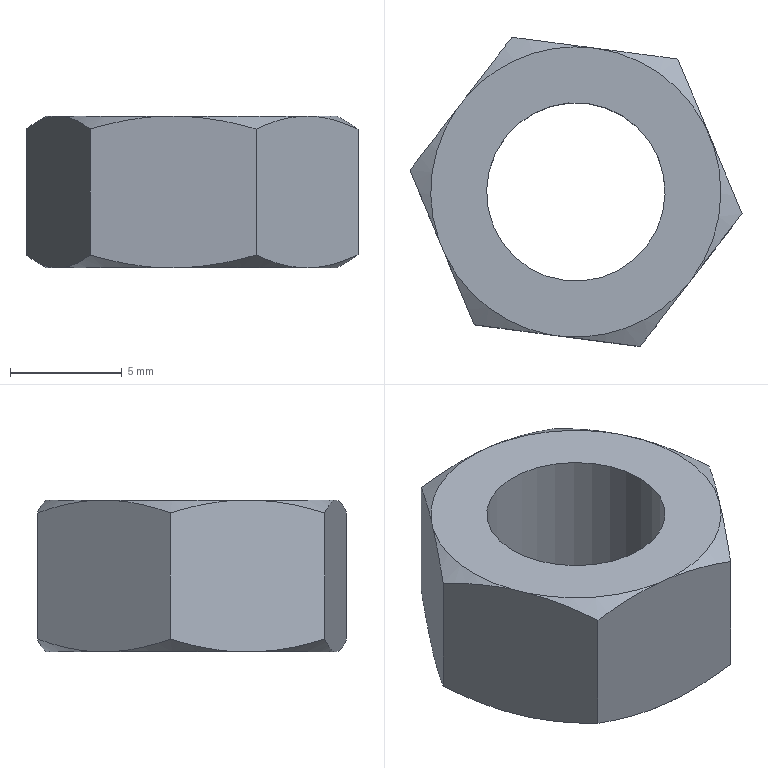Component | NX | 13_NUT | 1 solid | 19 faces | volume 649 mm3 | cone 10 | plane 8 | cylinder 1 | commonest cylinder face diameters 8 x1